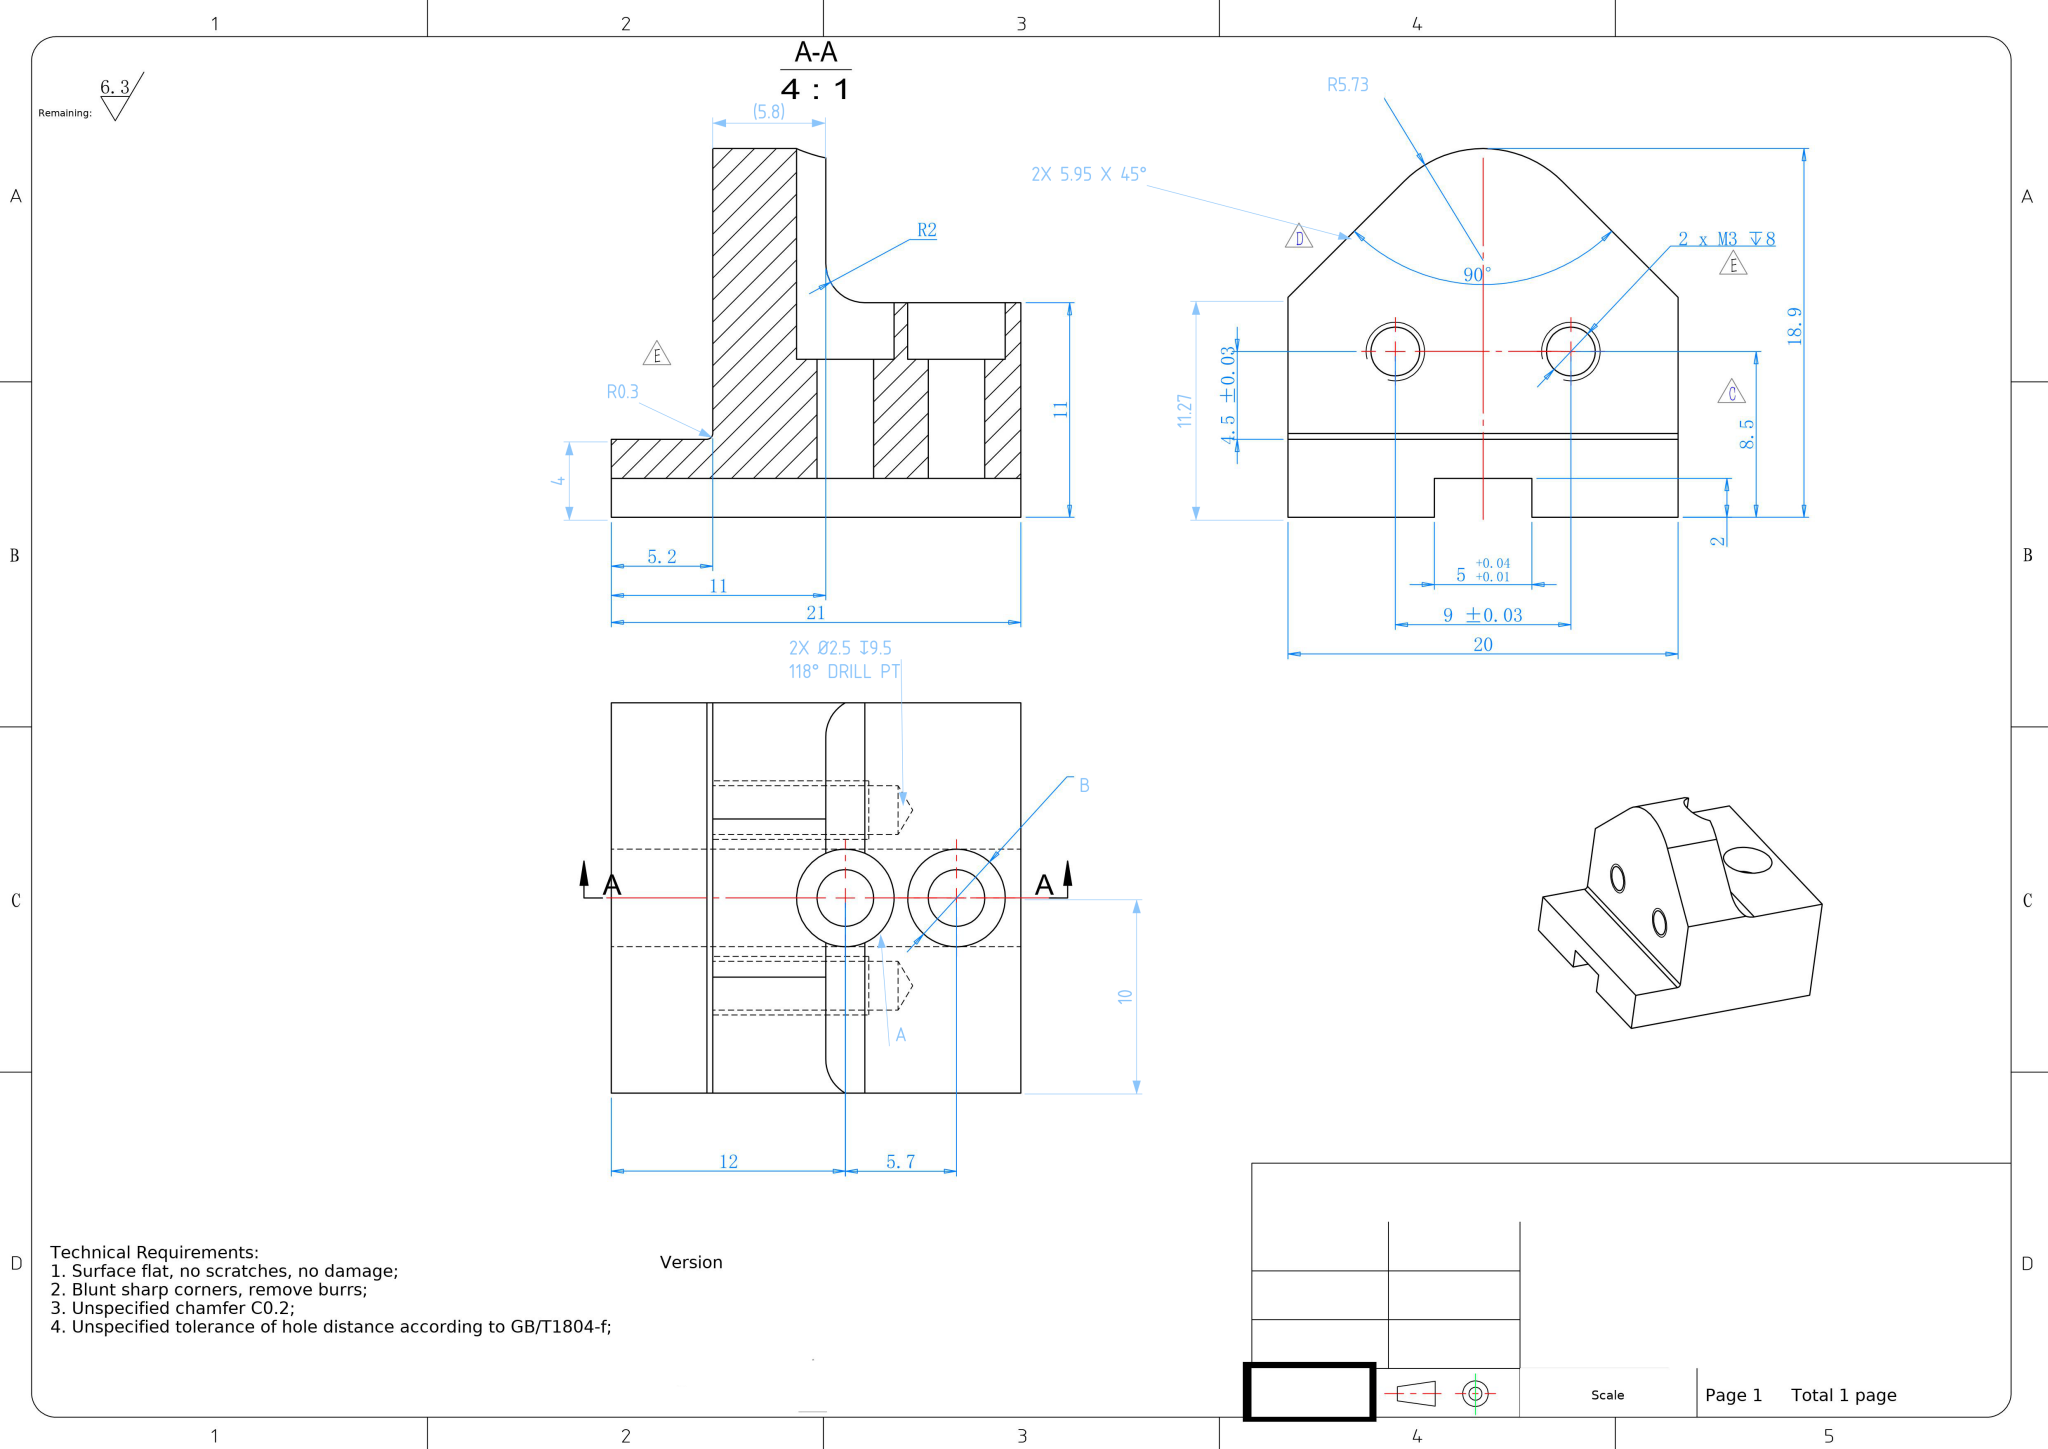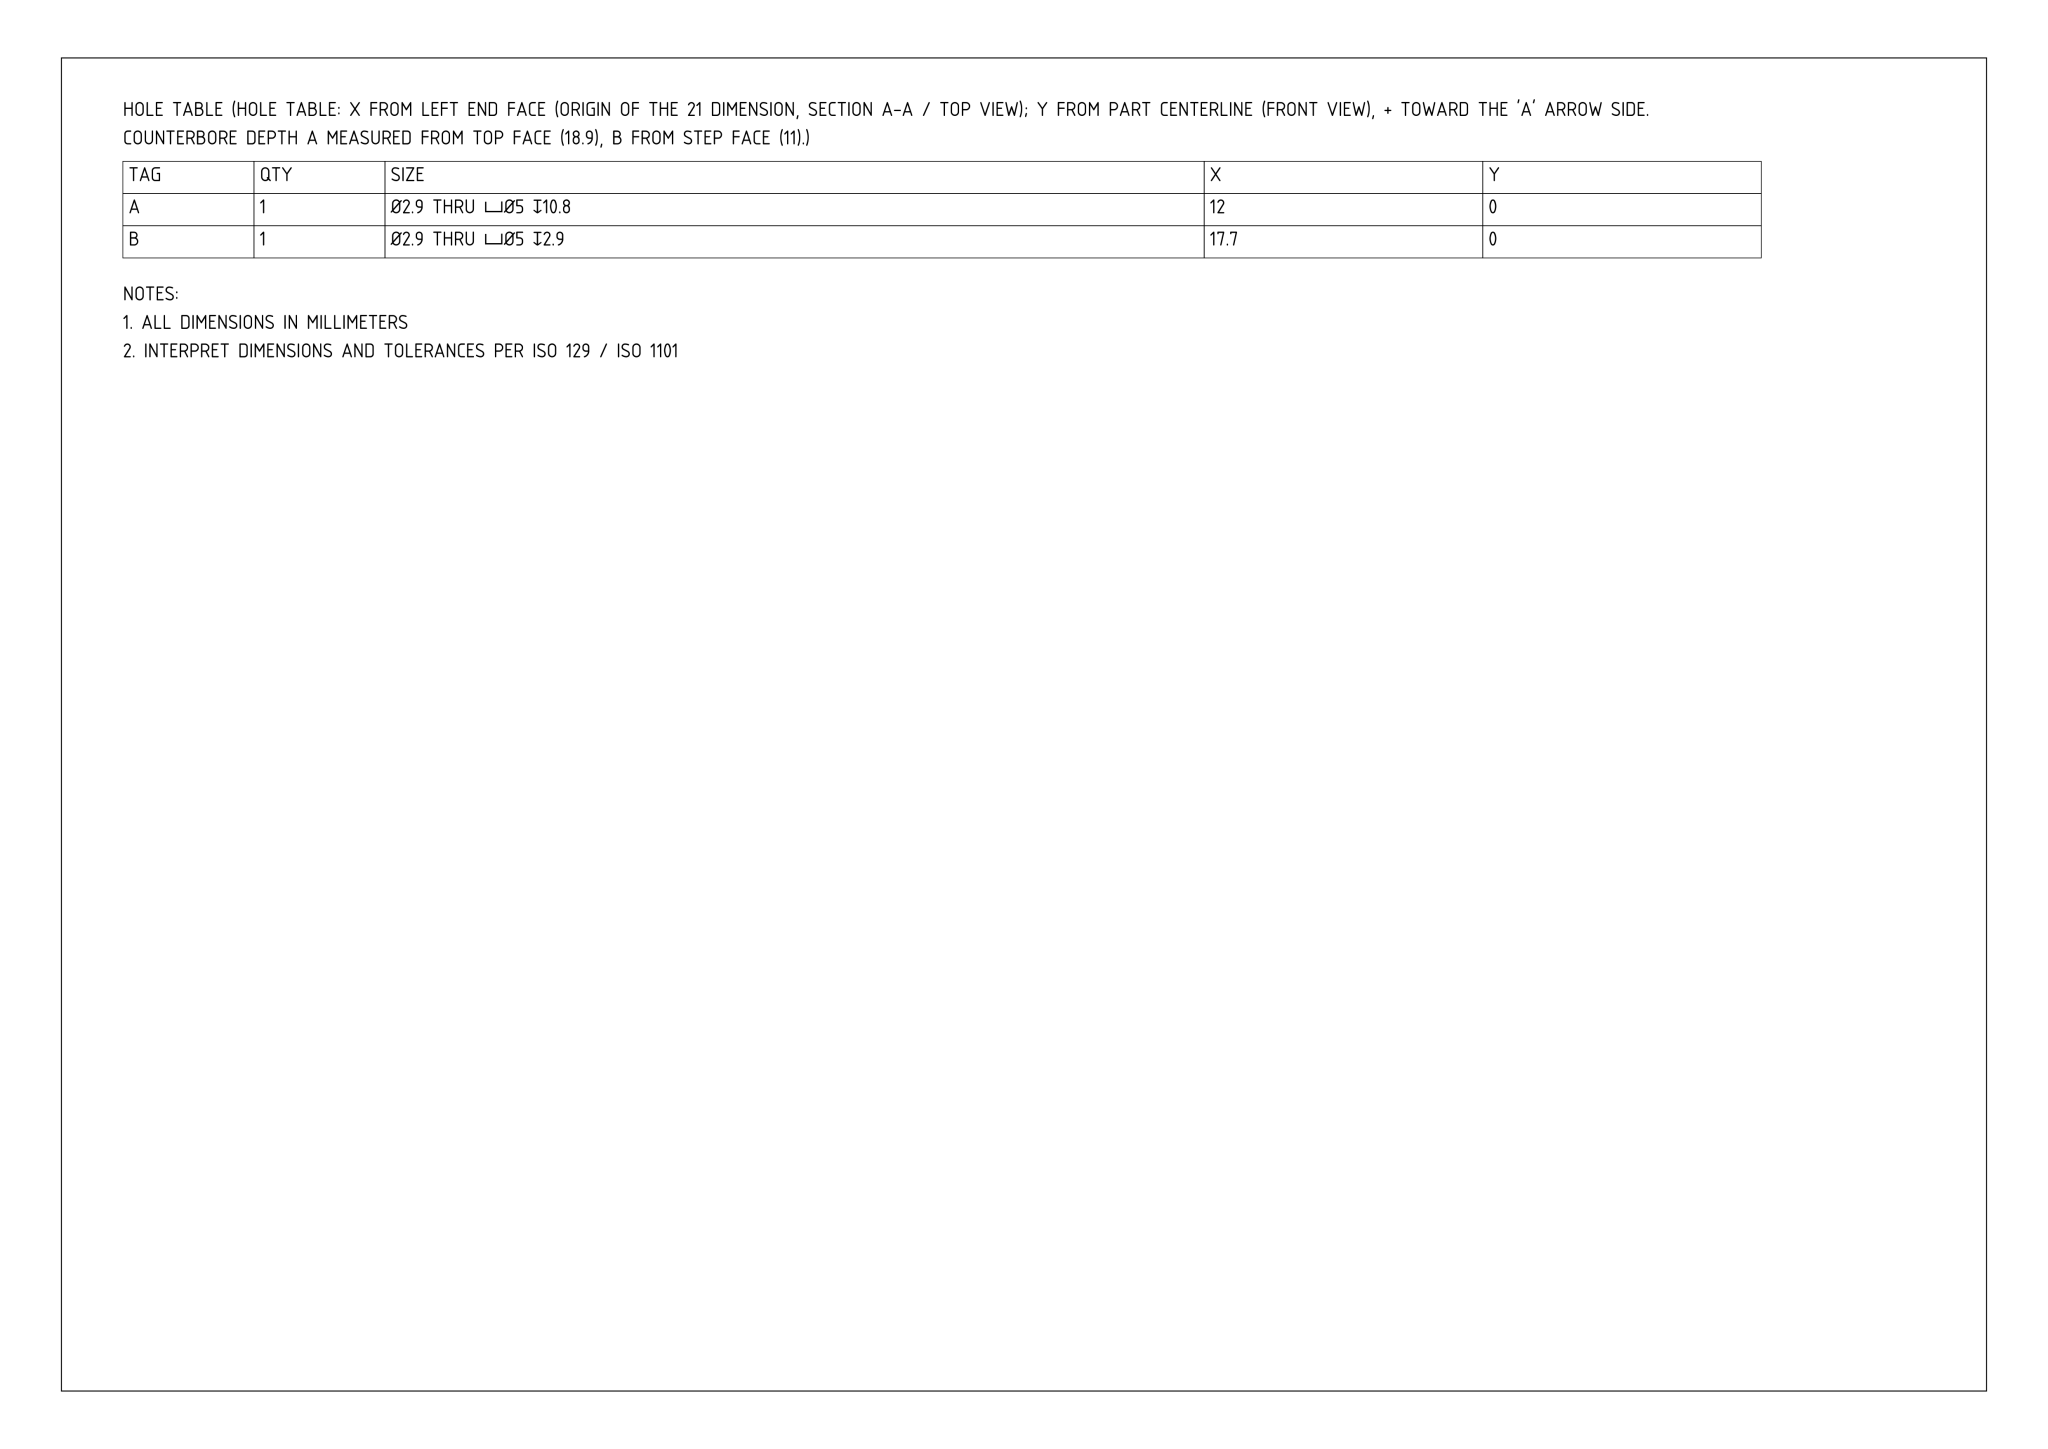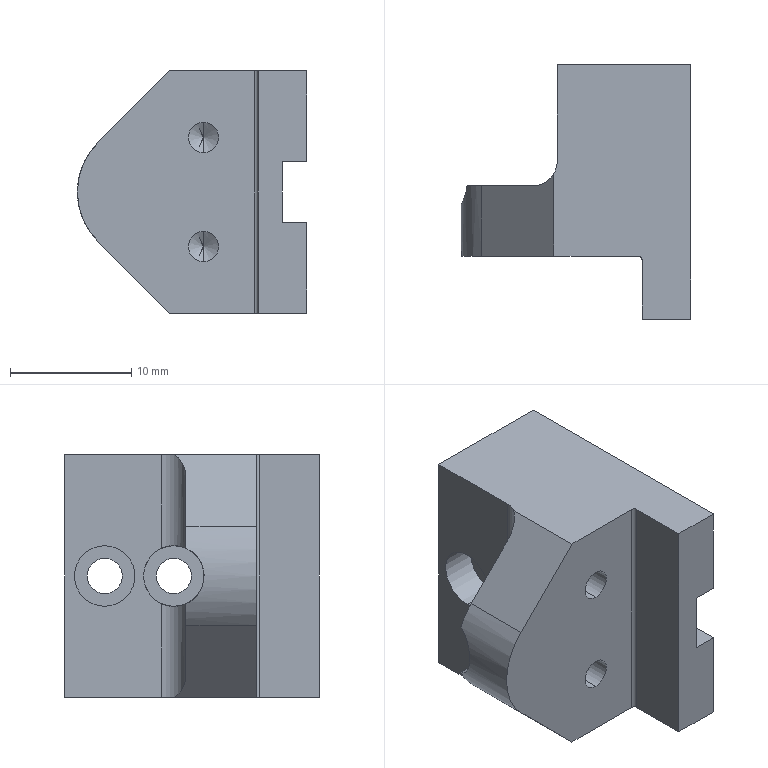Part | NX | mm | 1 solid | 38 faces | box 18.9 x 21 x 20 mm | volume 3937 mm3 | plane 18 | cylinder 16 | cone 4 | commonest cylinder face diameters 2.5 x4 5 x4 2.9 x4 4 x2 11.46 x1 0.6 x1